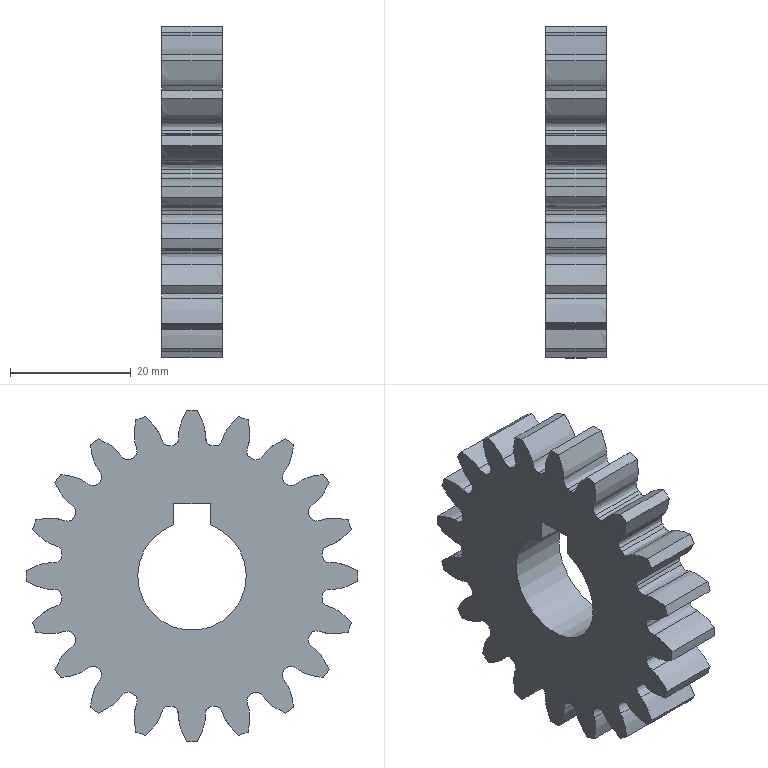Component | NX | GEAR_1 | 1 solid | 126 faces | volume 16561 mm3 | other 100 | cylinder 21 | plane 5 | commonest cylinder face diameters 43.75 x20 18 x1